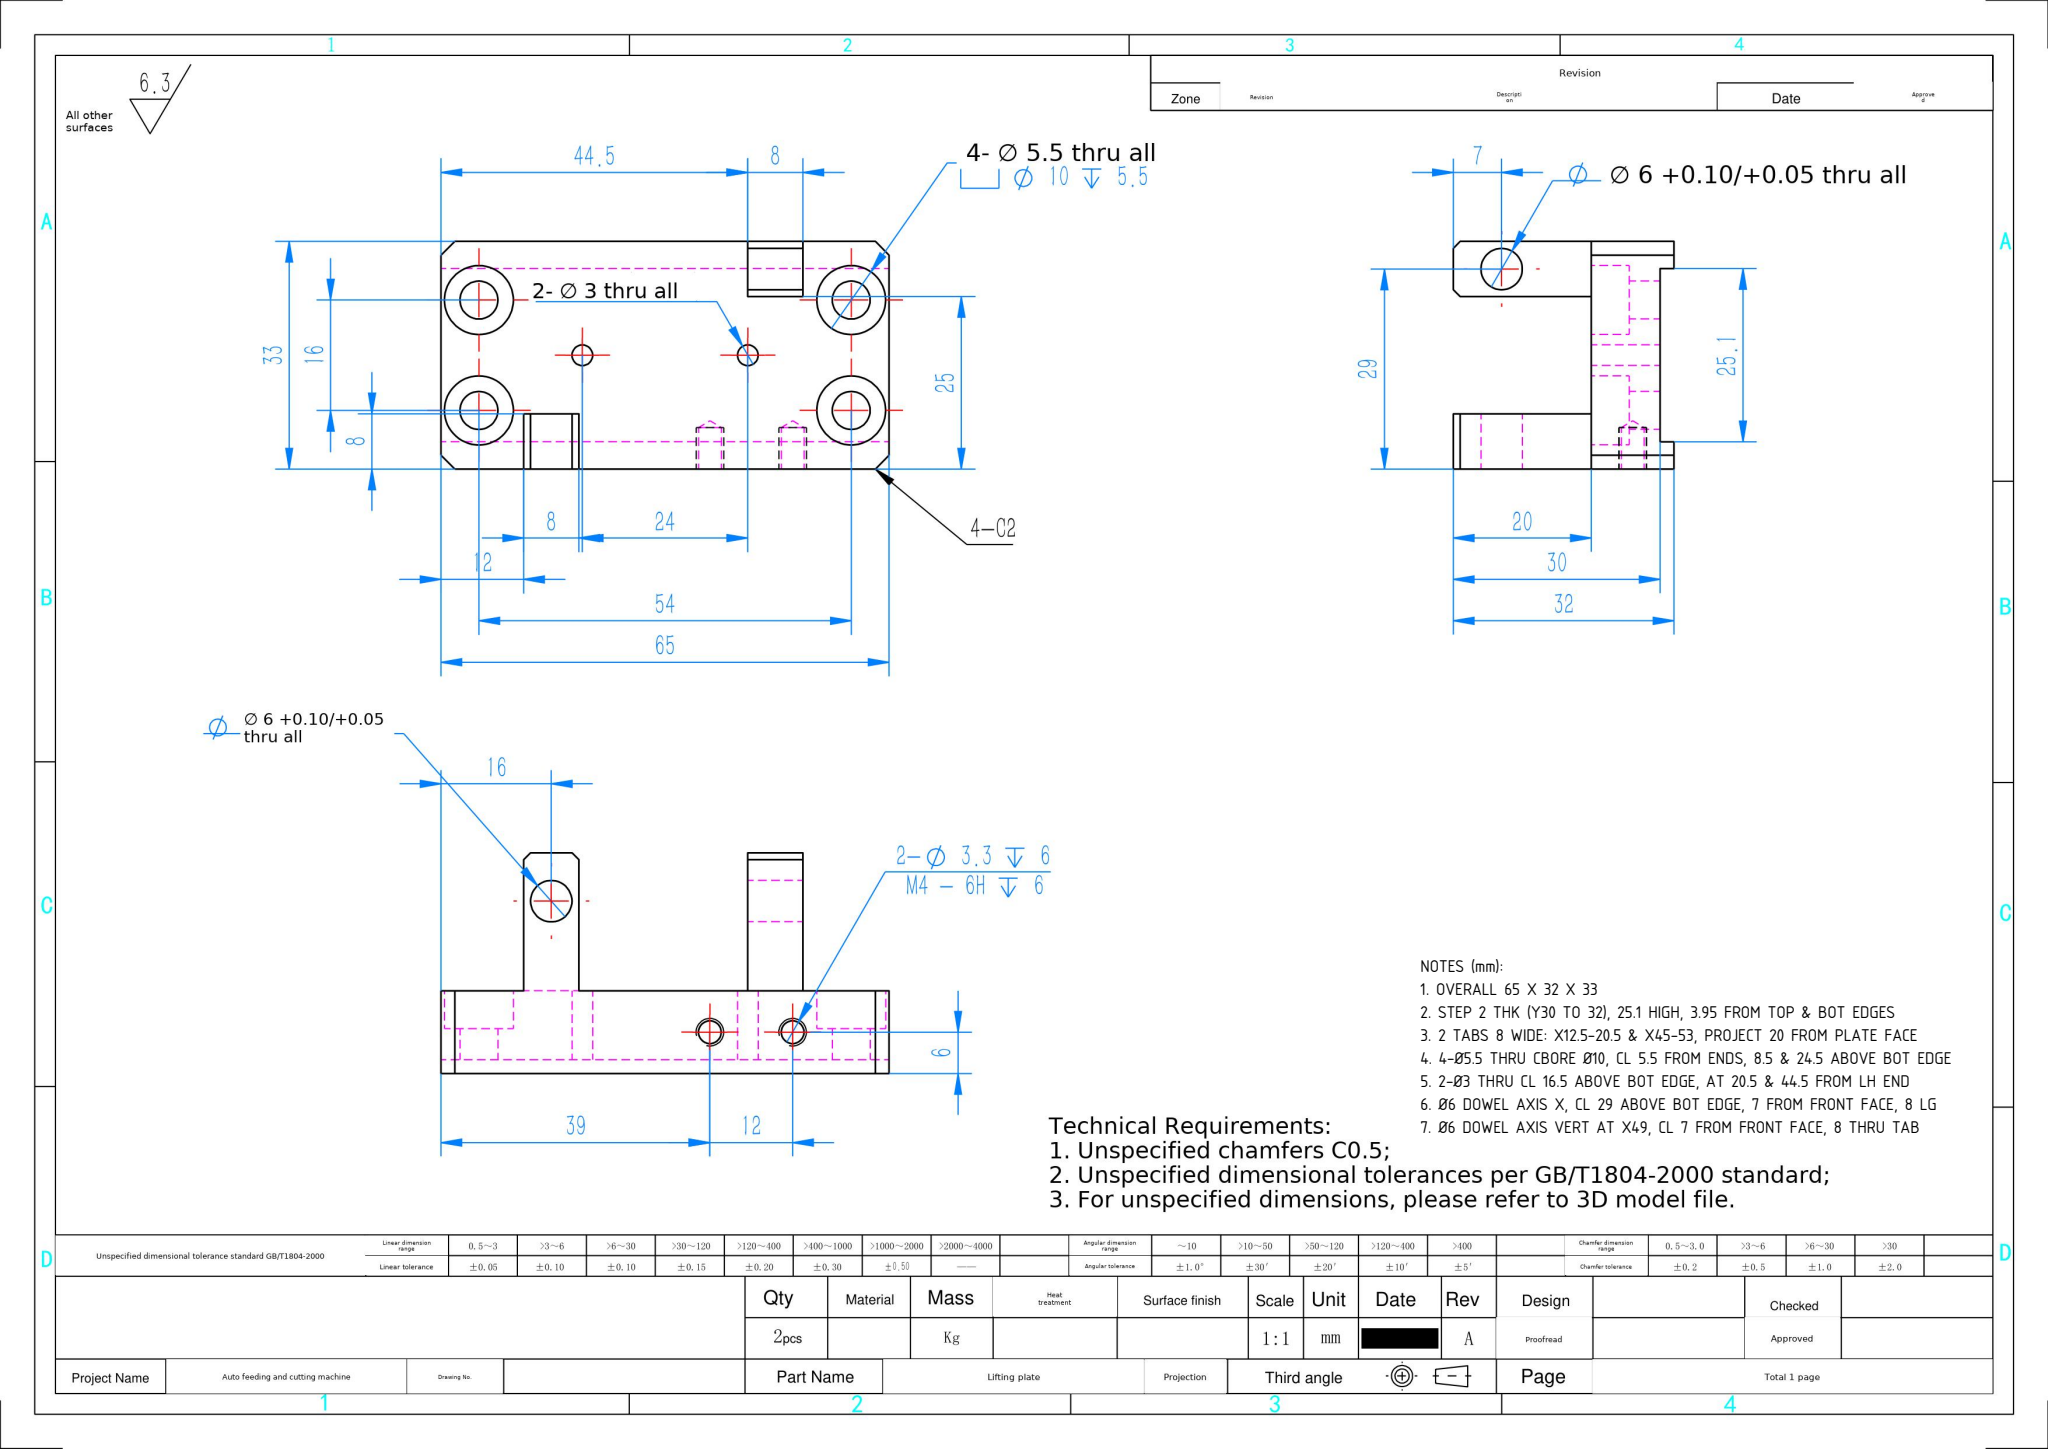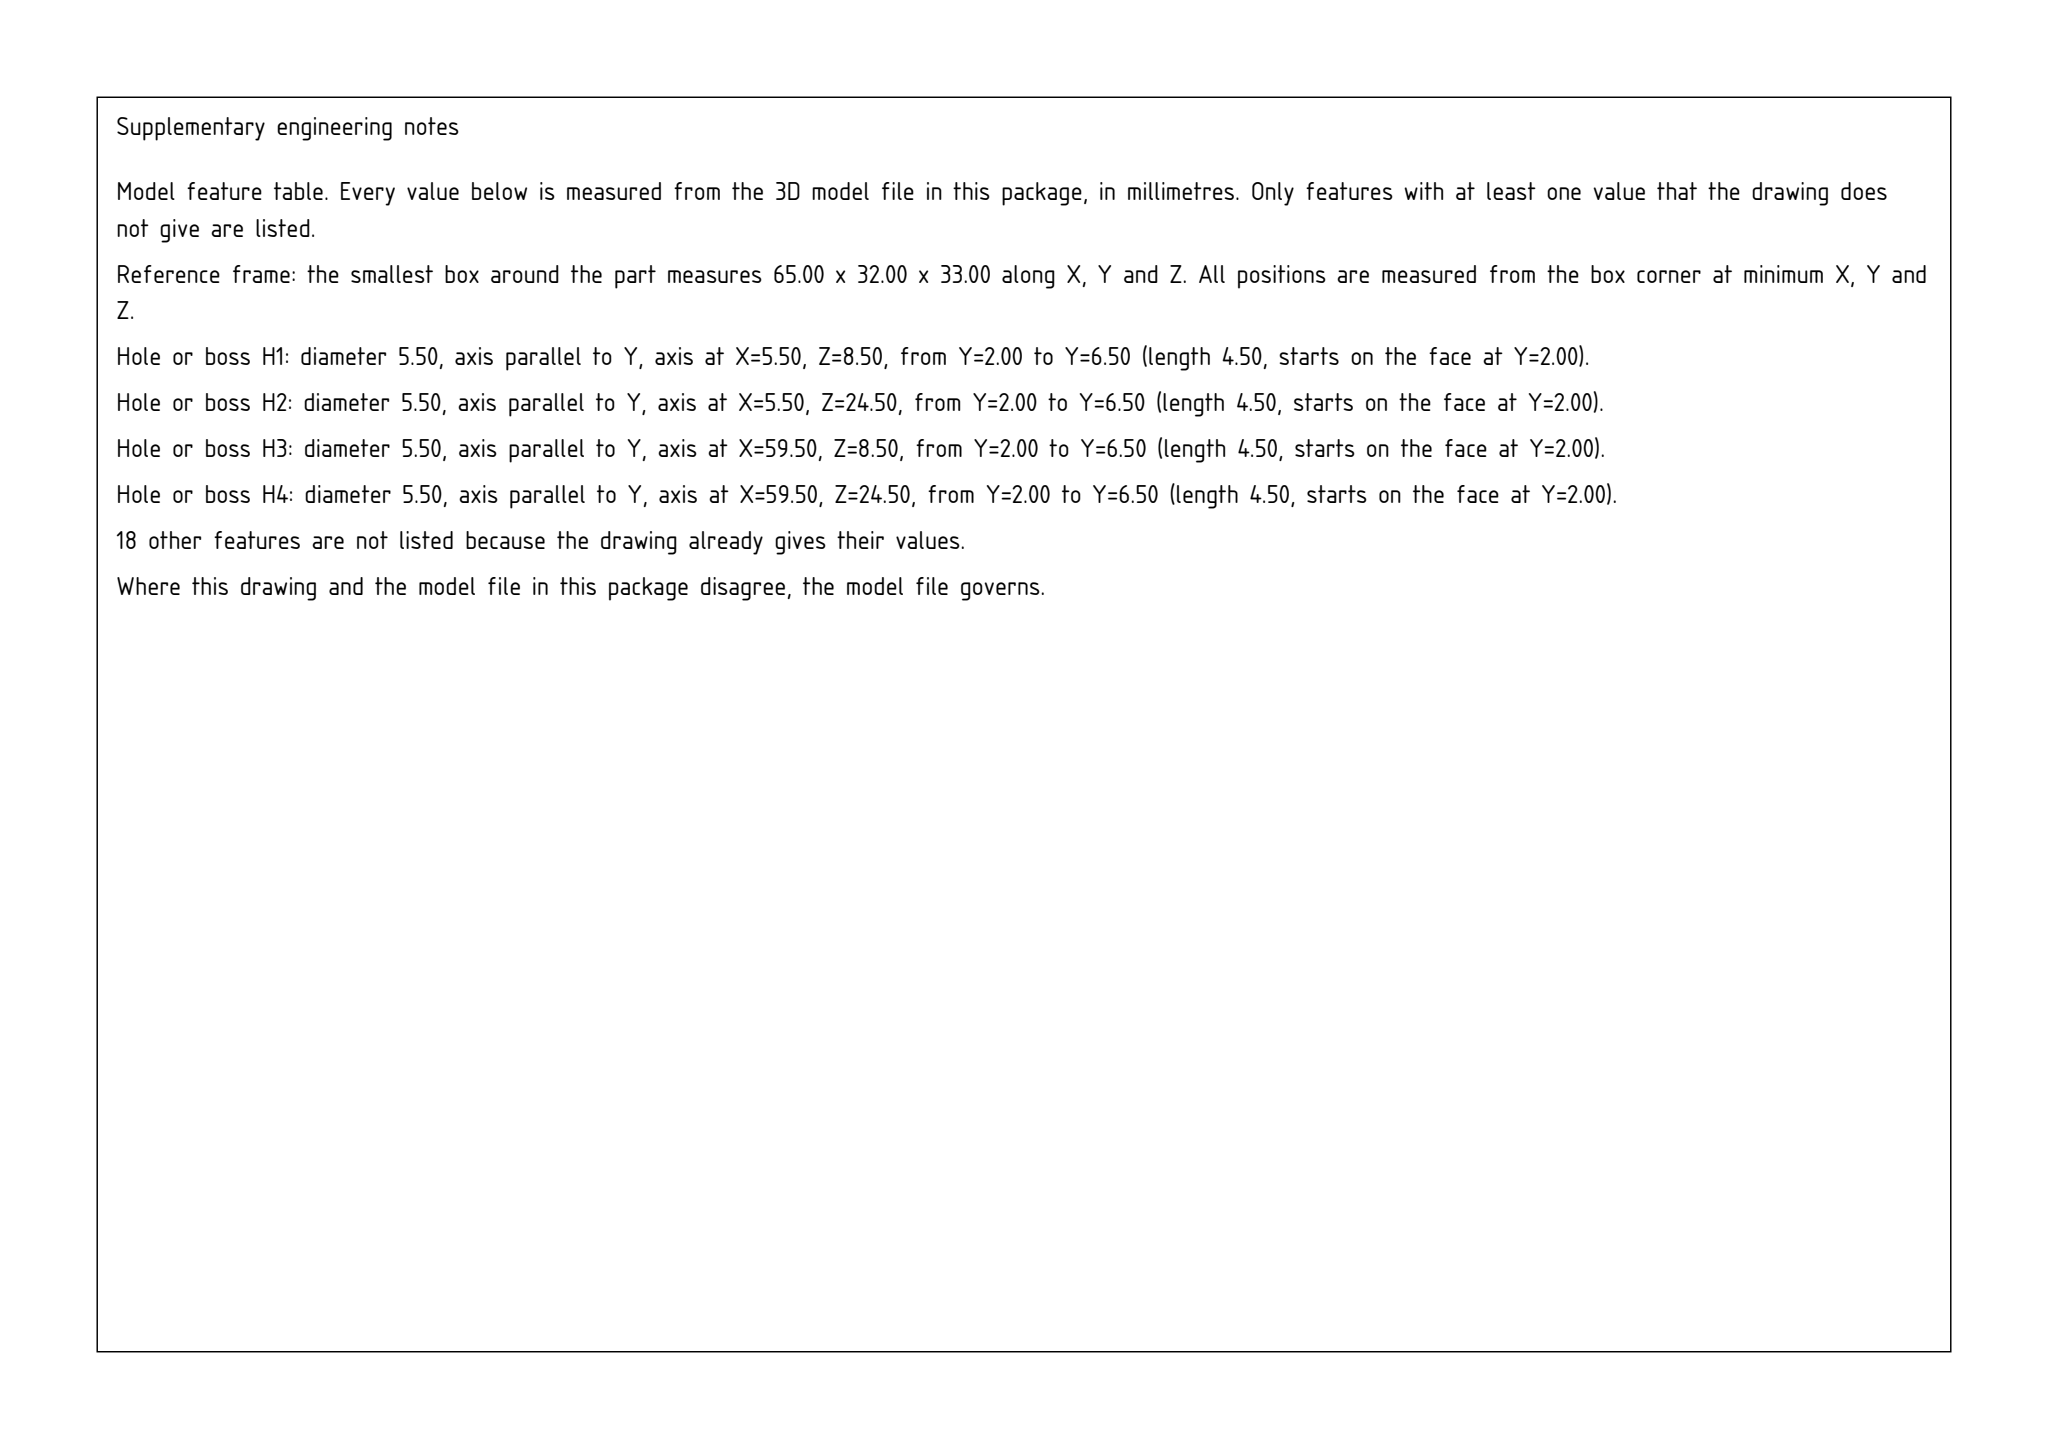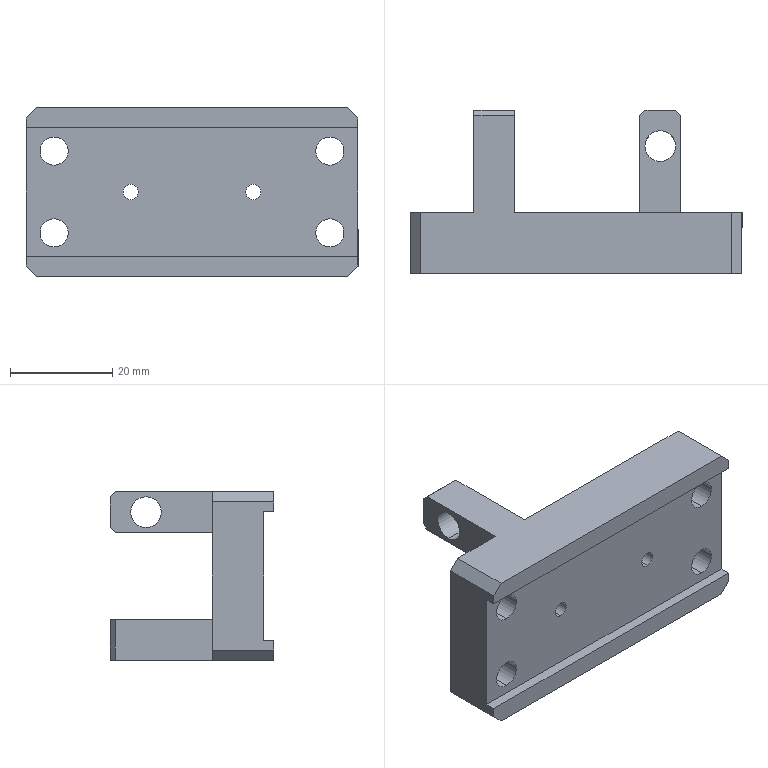Part | SolidWorks | mm | 1 solid | 62 faces | box 65 x 32 x 33 mm | volume 22067 mm3 | plane 30 | cylinder 28 | cone 4 | commonest cylinder face diameters 10 x8 5.5 x8 6 x4 3.3 x4 3 x4
Drawing notes:
OVERALL 65 X 32 X 33 | from the solid: bbox_xyz [65.0, 32.0, 33.0]
STEP 2 THK (Y30 TO 32), 25.1 HIGH, 3.95 FROM TOP & BOT EDGES | from the solid: y planes 0,2 (32-30=2); z planes 3.95 & 29.05 -> 25.1; 33-29.05=3.95
2 TABS 8 WIDE: X12.5-20.5 & X45-53, PROJECT 20 FROM PLATE FACE | from the solid: x planes 12.5,20.5,45,53; y planes 12 and 32 -> 20 projection
4-Ø5.5 THRU CBORE Ø10, CL 5.5 FROM ENDS, 8.5 & 24.5 ABOVE BOT EDGE | from the solid: cyl dia5.5 axis y at (5.5,8.5),(5.5,24.5),(59.5,8.5),(59.5,24.5); dia10 cbores same CL
2-Ø3 THRU CL 16.5 ABOVE BOT EDGE, AT 20.5 & 44.5 FROM LH END | from the solid: cyl dia3 axis y at (20.5,z16.5) and (44.5,z16.5), len 10
Ø6 DOWEL AXIS X, CL 29 ABOVE BOT EDGE, 7 FROM FRONT FACE, 8 LG | from the solid: cyl dia6 axis x at (y=25,z=29), len 8; bbox z=33, y=32 -> 32-25=7
Ø6 DOWEL AXIS VERT AT X49, CL 7 FROM FRONT FACE, 8 THRU TAB | from the solid: cyl dia6 axis z at (x=49,y=25), len 8 (z 25-33); 32-25=7
build123d program:
from build123d import *

# Parameters (mm, degrees)
SKETCH1_W                                       = 65
SKETCH1_H                                       = 33
BOSS_EXTRUDE1_DEPTH                             = 6
SKETCH2_W                                       = 65
SKETCH2_H                                       = 25.1
CUT_EXTRUDE1_DEPTH                              = 2
CHAMFER1_SIZE                                   = 2
M5_HEX_SOCKET_HEAD_CAP_SCREW_CBORE1_D           = 5.5
M5_HEX_SOCKET_HEAD_CAP_SCREW_CBORE1_CBORE_D     = 10
M5_HEX_SOCKET_HEAD_CAP_SCREW_CBORE1_CBORE_DEPTH = 5.5
SKETCH20_W                                      = 8
SKETCH20_H                                      = 8
BOSS_EXTRUDE2_DEPTH                             = 20
CHAMFER2_SIZE                                   = 1
F_3_0_3_DIAMETER_HOLE1_D                        = 3
M4_TAPPED_HOLE1_D                               = 3.3
M4_TAPPED_HOLE1_DEPTH                           = 6
M4_TAPPED_HOLE1_TIP                             = 0.9914
F_6_0_6_DIAMETER_HOLE2_D                        = 6
F_6_0_6_DIAMETER_HOLE2_ON_FACE_2_D              = 6


with BuildPart() as part:
    # Sketch1 → Boss-Extrude1 (new, symmetric)
    with BuildSketch(Plane(origin=(0, 0, 0), x_dir=(1, 0, 0), z_dir=(0, 1, 0))):
        Rectangle(SKETCH1_W, SKETCH1_H)
    extrude(amount=BOSS_EXTRUDE1_DEPTH, both=True)

    # Sketch2 → Cut-Extrude1 (cut)
    with BuildSketch(Plane.XZ.offset(6)):
        Rectangle(SKETCH2_W, SKETCH2_H)
    extrude(amount=-CUT_EXTRUDE1_DEPTH, mode=Mode.SUBTRACT)

    # Chamfer1
    chamfer1_edges = [part.edges().sort_by_distance(p)[0] for p in [
        (32.5, 0, 16.5),
        (-32.5, 0, 16.5),
        (-32.5, 0, -16.5),
        (32.5, 0, -16.5),
    ]]
    chamfer(chamfer1_edges, length=CHAMFER1_SIZE)

    # M5 Hex Socket Head Cap Screw CBORE1 (through all)
    with Locations(Plane(origin=(0, 6, 0), x_dir=(1, 0, 0), z_dir=(0, 1, 0))):
        with Locations((-27, 8), (27, 8), (27, -8), (-27, -8)):
            CounterBoreHole(M5_HEX_SOCKET_HEAD_CAP_SCREW_CBORE1_D / 2, M5_HEX_SOCKET_HEAD_CAP_SCREW_CBORE1_CBORE_D / 2, M5_HEX_SOCKET_HEAD_CAP_SCREW_CBORE1_CBORE_DEPTH)

    # Sketch20 → Boss-Extrude2 (add)
    with BuildSketch(Plane(origin=(0, 6, 0), x_dir=(1, 0, 0), z_dir=(0, 1, 0))):
        with Locations((-16, -12.5)):
            Rectangle(SKETCH20_W, SKETCH20_H)
        with Locations((16.5, 12.5)):
            Rectangle(SKETCH20_W, SKETCH20_H)
    extrude(amount=BOSS_EXTRUDE2_DEPTH)

    # Chamfer2
    chamfer2_edges = [part.edges().sort_by_distance(p)[0] for p in [
        (-16, 26, 8.5),
        (-16, 26, 16.5),
        (20.5, 26, -12.5),
        (12.5, 26, -12.5),
    ]]
    chamfer(chamfer2_edges, length=CHAMFER2_SIZE)

    # 3.0 _3_ Diameter Hole1 (through all)
    with Locations(Plane(origin=(0, -4, 0), x_dir=(-1, 0, 0), z_dir=(0, -1, 0))):
        with Locations((12, 0), (-12, 0)):
            Hole(F_3_0_3_DIAMETER_HOLE1_D / 2)

    # M4 Tapped Hole1
    with Locations(Plane(origin=(0, 0, -16.5), x_dir=(-1, 0, 0), z_dir=(0, 0, -1))):
        with Locations((18.5, 0), (6.5, 0)):
            Hole(M4_TAPPED_HOLE1_D / 2, depth=M4_TAPPED_HOLE1_DEPTH)
            with Locations((0, 0, -(M4_TAPPED_HOLE1_DEPTH + M4_TAPPED_HOLE1_TIP / 2))):  # 118° drill point
                Cone(0, M4_TAPPED_HOLE1_D / 2, M4_TAPPED_HOLE1_TIP, mode=Mode.SUBTRACT)

    # 6.0 _6_ Diameter Hole2 (through all)
    with Locations(Plane(origin=(-12, 19, 12.5), x_dir=(0, 0, 1), z_dir=(1, 0, 0))):
        with Locations((0, 0)):
            Hole(F_6_0_6_DIAMETER_HOLE2_D / 2)

    # 6.0 _6_ Diameter Hole2 on face 2 (through all)
    with Locations(Plane(origin=(16.5, 19, -8.5), x_dir=(1, 0, 0), z_dir=(0, 0, 1))):
        with Locations((0, 0)):
            Hole(F_6_0_6_DIAMETER_HOLE2_ON_FACE_2_D / 2)


solid = part.part